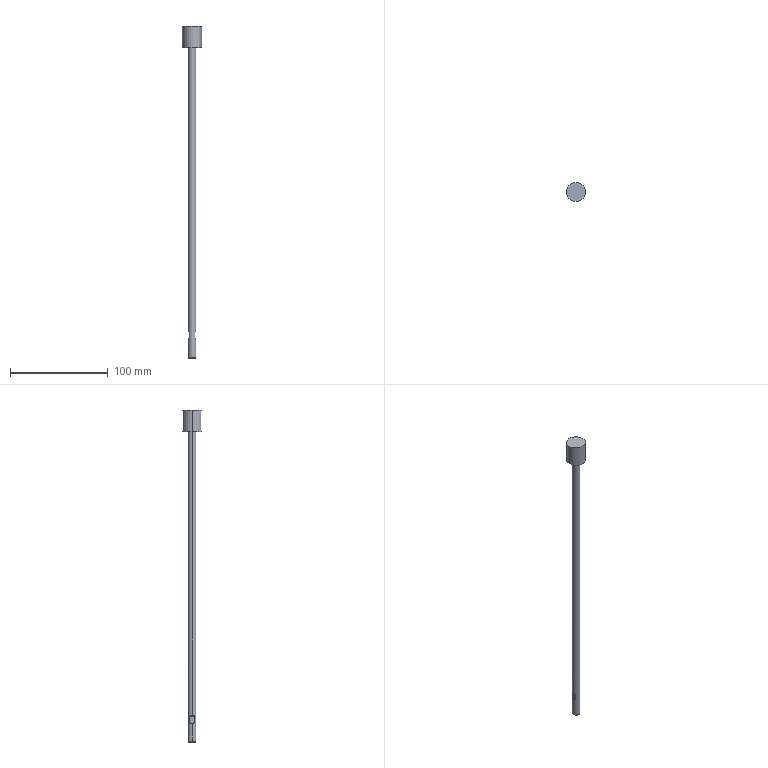Component | SolidWorks | F01AE00111-A2000-21TopEdgeAssembly-1_MA20x250SU(0)+(CS1-M-2)-1_20UMA250 Rod-1 | 1 solid | 15 faces | box 19.5 x 19.5 x 339 mm | volume 22445 mm3 | plane 9 | cylinder 4 | cone 2 | commonest cylinder face diameters 19.5 x2 8 x2
build123d program:
from build123d import *

# Parameters (mm, degrees)
CUT_EXTRUDE1_DEPTH      = 3
CUT_EXTRUDE1_DEPTH_BACK = 3


with BuildPart() as part:
    # Sketch1 → Revolve1 (revolve)
    with BuildSketch(Plane.XY, mode=Mode.PRIVATE) as revolve1_sk:
        Polygon((0, 0), (0, 3.233), (0.767, 4), (317, 4), (317, 9.75), (339, 9.75), (339, 0), align=None)
    revolve(revolve1_sk.sketch.rotate(Axis((339, 0, 0), (-1, 0, 0)), 270), axis=Axis((339, 0, 0), (-1, 0, 0)))

    # Sketch2 → Cut-Extrude1 (cut, two sides: drawn at the far end of the back side and taken through both)
    with BuildSketch(Plane(origin=(0, 0, 0), x_dir=(1, 0, 0), z_dir=(0, 1, 0)).offset(-CUT_EXTRUDE1_DEPTH_BACK)):
        Polygon((-5, 12), (-5, -12), (35.4, -12), (26.4, -3), (20, -3), (18, -5), (18, -10), (-3, -10), (-3, 10), (18, 10), (18, 5), (20, 3), (26.4, 3), (35.4, 12), align=None)
    extrude(amount=CUT_EXTRUDE1_DEPTH + CUT_EXTRUDE1_DEPTH_BACK, mode=Mode.SUBTRACT)


solid = part.part

# Placed as in the assembly
solid = solid.moved(Location((-109.352, 82.548, -371.975), (0, -90, 0)))
STEP:
#1=COLOUR_RGB('',0.7922,0.8196,0.9333);
#2=FILL_AREA_STYLE_COLOUR('',#1);
#3=FILL_AREA_STYLE('',(#2));
#4=SURFACE_STYLE_FILL_AREA(#3);
#5=SURFACE_SIDE_STYLE('',(#4));
#6=SURFACE_STYLE_USAGE(.BOTH.,#5);
#7=PRESENTATION_STYLE_ASSIGNMENT((#6));
#8=CARTESIAN_POINT('',(-3.921,3.25,-1.298));
#9=VERTEX_POINT('',#8);
#10=CARTESIAN_POINT('',(-4.689,3.25,-1.298));
#11=VERTEX_POINT('',#10);
#12=CARTESIAN_POINT('',(-4.305,3.25,-1.298));
#13=DIRECTION('',(-0.,-0.,-1.));
#14=DIRECTION('',(1.,0.,0.));
#15=AXIS2_PLACEMENT_3D('',#12,#13,#14);
#16=CIRCLE('',#15,0.3839);
#17=EDGE_CURVE('',#9,#11,#16,.T.);
#18=ORIENTED_EDGE('',*,*,#17,.T.);
#19=CARTESIAN_POINT('',(-4.689,3.25,-2.164));
#20=VERTEX_POINT('',#19);
#21=CARTESIAN_POINT('',(-4.689,3.25,-1.298));
#22=DIRECTION('',(-0.,-0.,-1.));
#23=VECTOR('',#22,39.37);
#24=LINE('',#21,#23);
#25=EDGE_CURVE('',#11,#20,#24,.T.);
#26=ORIENTED_EDGE('',*,*,#25,.T.);
#27=CARTESIAN_POINT('',(-3.921,3.25,-2.164));
#28=VERTEX_POINT('',#27);
#29=CARTESIAN_POINT('',(-4.305,3.25,-2.164));
#30=DIRECTION('',(-0.,-0.,-1.));
#31=DIRECTION('',(1.,0.,0.));
#32=AXIS2_PLACEMENT_3D('',#29,#30,#31);
#33=CIRCLE('',#32,0.3839);
#34=EDGE_CURVE('',#28,#20,#33,.T.);
#35=ORIENTED_EDGE('',*,*,#34,.F.);
#36=CARTESIAN_POINT('',(-3.921,3.25,-1.298));
#37=DIRECTION('',(-0.,-0.,-1.));
#38=VECTOR('',#37,39.37);
#39=LINE('',#36,#38);
#40=EDGE_CURVE('',#9,#28,#39,.T.);
#41=ORIENTED_EDGE('',*,*,#40,.F.);
#42=EDGE_LOOP('',(#18,#26,#35,#41));
#43=FACE_OUTER_BOUND('',#42,.T.);
#44=CARTESIAN_POINT('',(-4.305,3.25,-1.298));
#45=DIRECTION('',(-0.,-0.,-1.));
#46=DIRECTION('',(1.,0.,0.));
#47=AXIS2_PLACEMENT_3D('',#44,#45,#46);
#48=CYLINDRICAL_SURFACE('',#47,0.3839);
#49=ADVANCED_FACE('',(#43),#48,.T.);
#50=CARTESIAN_POINT('',(-4.148,3.25,-2.164));
#51=VERTEX_POINT('',#50);
#52=CARTESIAN_POINT('',(-4.463,3.25,-2.164));
#53=VERTEX_POINT('',#52);
#54=CARTESIAN_POINT('',(-4.305,3.25,-2.164));
#55=DIRECTION('',(-0.,-0.,-1.));
#56=DIRECTION('',(1.,0.,0.));
#57=AXIS2_PLACEMENT_3D('',#54,#55,#56);
#58=CIRCLE('',#57,0.1575);
#59=EDGE_CURVE('',#51,#53,#58,.T.);
#60=ORIENTED_EDGE('',*,*,#59,.T.);
#61=CARTESIAN_POINT('',(-4.463,3.25,-13.566));
#62=VERTEX_POINT('',#61);
#63=CARTESIAN_POINT('',(-4.463,3.25,-1.298));
#64=DIRECTION('',(-0.,-0.,-1.));
#65=VECTOR('',#64,39.37);
#66=LINE('',#63,#65);
#67=EDGE_CURVE('',#53,#62,#66,.T.);
#68=ORIENTED_EDGE('',*,*,#67,.T.);
#69=CARTESIAN_POINT('',(-4.423,3.146,-13.605));
#70=VERTEX_POINT('',#69);
#71=CARTESIAN_POINT('',(-4.463,3.25,-13.566));
#72=CARTESIAN_POINT('',(-4.463,3.211,-13.566));
#73=CARTESIAN_POINT('',(-4.449,3.175,-13.58));
#74=CARTESIAN_POINT('',(-4.423,3.146,-13.605));
#75=(BOUNDED_CURVE()B_SPLINE_CURVE(3,(#71,#72,#73,#74),.UNSPECIFIED.,.F.,.T.)B_SPLINE_CURVE_WITH_KNOTS((4,4),(3.142,3.864),.UNSPECIFIED.)CURVE()GEOMETRIC_REPRESENTATION_ITEM()RATIONAL_B_SPLINE_CURVE((1.,0.9569,0.9569,1.))REPRESENTATION_ITEM(''));
#76=EDGE_CURVE('',#62,#70,#75,.T.);
#77=ORIENTED_EDGE('',*,*,#76,.T.);
#78=CARTESIAN_POINT('',(-4.423,3.146,-13.857));
#79=VERTEX_POINT('',#78);
#80=CARTESIAN_POINT('',(-4.423,3.146,-1.298));
#81=DIRECTION('',(-0.,-0.,-1.));
#82=VECTOR('',#81,39.37);
#83=LINE('',#80,#82);
#84=EDGE_CURVE('',#70,#79,#83,.T.);
#85=ORIENTED_EDGE('',*,*,#84,.T.);
#86=CARTESIAN_POINT('',(-4.463,3.25,-13.897));
#87=VERTEX_POINT('',#86);
#88=CARTESIAN_POINT('',(-4.423,3.146,-13.857));
#89=CARTESIAN_POINT('',(-4.449,3.175,-13.883));
#90=CARTESIAN_POINT('',(-4.463,3.211,-13.897));
#91=CARTESIAN_POINT('',(-4.463,3.25,-13.897));
#92=(BOUNDED_CURVE()B_SPLINE_CURVE(3,(#88,#89,#90,#91),.UNSPECIFIED.,.F.,.T.)B_SPLINE_CURVE_WITH_KNOTS((4,4),(5.56,6.283),.UNSPECIFIED.)CURVE()GEOMETRIC_REPRESENTATION_ITEM()RATIONAL_B_SPLINE_CURVE((1.,0.9569,0.9569,1.))REPRESENTATION_ITEM(''));
#93=EDGE_CURVE('',#79,#87,#92,.T.);
#94=ORIENTED_EDGE('',*,*,#93,.T.);
#95=CARTESIAN_POINT('',(-4.463,3.25,-14.614));
#96=VERTEX_POINT('',#95);
#97=CARTESIAN_POINT('',(-4.463,3.25,-1.298));
#98=DIRECTION('',(-0.,-0.,-1.));
#99=VECTOR('',#98,39.37);
#100=LINE('',#97,#99);
#101=EDGE_CURVE('',#87,#96,#100,.T.);
#102=ORIENTED_EDGE('',*,*,#101,.T.);
#103=CARTESIAN_POINT('',(-4.148,3.25,-14.614));
#104=VERTEX_POINT('',#103);
#105=CARTESIAN_POINT('',(-4.305,3.25,-14.614));
#106=DIRECTION('',(-0.,-0.,-1.));
#107=DIRECTION('',(1.,0.,0.));
#108=AXIS2_PLACEMENT_3D('',#105,#106,#107);
#109=CIRCLE('',#108,0.1575);
#110=EDGE_CURVE('',#104,#96,#109,.T.);
#111=ORIENTED_EDGE('',*,*,#110,.F.);
#112=CARTESIAN_POINT('',(-4.148,3.25,-13.897));
#113=VERTEX_POINT('',#112);
#114=CARTESIAN_POINT('',(-4.148,3.25,-1.298));
#115=DIRECTION('',(-0.,-0.,-1.));
#116=VECTOR('',#115,39.37);
#117=LINE('',#114,#116);
#118=EDGE_CURVE('',#113,#104,#117,.T.);
#119=ORIENTED_EDGE('',*,*,#118,.F.);
#120=CARTESIAN_POINT('',(-4.187,3.146,-13.857));
#121=VERTEX_POINT('',#120);
#122=CARTESIAN_POINT('',(-4.148,3.25,-13.897));
#123=CARTESIAN_POINT('',(-4.148,3.211,-13.897));
#124=CARTESIAN_POINT('',(-4.161,3.175,-13.883));
#125=CARTESIAN_POINT('',(-4.187,3.146,-13.857));
#126=(BOUNDED_CURVE()B_SPLINE_CURVE(3,(#122,#123,#124,#125),.UNSPECIFIED.,.F.,.T.)B_SPLINE_CURVE_WITH_KNOTS((4,4),(0.,0.7227),.UNSPECIFIED.)CURVE()GEOMETRIC_REPRESENTATION_ITEM()RATIONAL_B_SPLINE_CURVE((1.,0.9569,0.9569,1.))REPRESENTATION_ITEM(''));
#127=EDGE_CURVE('',#113,#121,#126,.T.);
#128=ORIENTED_EDGE('',*,*,#127,.T.);
#129=CARTESIAN_POINT('',(-4.187,3.146,-13.605));
#130=VERTEX_POINT('',#129);
#131=CARTESIAN_POINT('',(-4.187,3.146,-1.298));
#132=DIRECTION('',(0.,0.,1.));
#133=VECTOR('',#132,39.37);
#134=LINE('',#131,#133);
#135=EDGE_CURVE('',#121,#130,#134,.T.);
#136=ORIENTED_EDGE('',*,*,#135,.T.);
#137=CARTESIAN_POINT('',(-4.148,3.25,-13.566));
#138=VERTEX_POINT('',#137);
#139=CARTESIAN_POINT('',(-4.187,3.146,-13.605));
#140=CARTESIAN_POINT('',(-4.161,3.175,-13.58));
#141=CARTESIAN_POINT('',(-4.148,3.211,-13.566));
#142=CARTESIAN_POINT('',(-4.148,3.25,-13.566));
#143=(BOUNDED_CURVE()B_SPLINE_CURVE(3,(#139,#140,#141,#142),.UNSPECIFIED.,.F.,.T.)B_SPLINE_CURVE_WITH_KNOTS((4,4),(2.419,3.142),.UNSPECIFIED.)CURVE()GEOMETRIC_REPRESENTATION_ITEM()RATIONAL_B_SPLINE_CURVE((1.,0.9569,0.9569,1.))REPRESENTATION_ITEM(''));
#144=EDGE_CURVE('',#130,#138,#143,.T.);
#145=ORIENTED_EDGE('',*,*,#144,.T.);
#146=CARTESIAN_POINT('',(-4.148,3.25,-1.298));
#147=DIRECTION('',(-0.,-0.,-1.));
#148=VECTOR('',#147,39.37);
#149=LINE('',#146,#148);
#150=EDGE_CURVE('',#51,#138,#149,.T.);
#151=ORIENTED_EDGE('',*,*,#150,.F.);
#152=EDGE_LOOP('',(#60,#68,#77,#85,#94,#102,#111,#119,#128,#136,#145,#151));
#153=FACE_OUTER_BOUND('',#152,.T.);
#154=CARTESIAN_POINT('',(-4.305,3.25,-1.298));
#155=DIRECTION('',(-0.,-0.,-1.));
#156=DIRECTION('',(1.,0.,0.));
#157=AXIS2_PLACEMENT_3D('',#154,#155,#156);
#158=CYLINDRICAL_SURFACE('',#157,0.1575);
#159=ADVANCED_FACE('',(#153),#158,.T.);
#160=CARTESIAN_POINT('',(-4.178,3.25,-14.645));
#161=VERTEX_POINT('',#160);
#162=CARTESIAN_POINT('',(-4.432,3.25,-14.645));
#163=VERTEX_POINT('',#162);
#164=CARTESIAN_POINT('',(-4.305,3.25,-14.645));
#165=DIRECTION('',(-0.,-0.,-1.));
#166=DIRECTION('',(1.,0.,0.));
#167=AXIS2_PLACEMENT_3D('',#164,#165,#166);
#168=CIRCLE('',#167,0.1273);
#169=EDGE_CURVE('',#161,#163,#168,.T.);
#170=ORIENTED_EDGE('',*,*,#169,.F.);
#171=CARTESIAN_POINT('',(-4.148,3.25,-14.614));
#172=DIRECTION('',(0.7071,-0.,0.7071));
#173=VECTOR('',#172,39.37);
#174=LINE('',#171,#173);
#175=EDGE_CURVE('',#161,#104,#174,.T.);
#176=ORIENTED_EDGE('',*,*,#175,.T.);
#177=ORIENTED_EDGE('',*,*,#110,.T.);
#178=CARTESIAN_POINT('',(-4.463,3.25,-14.614));
#179=DIRECTION('',(-0.7071,0.,0.7071));
#180=VECTOR('',#179,39.37);
#181=LINE('',#178,#180);
#182=EDGE_CURVE('',#163,#96,#181,.T.);
#183=ORIENTED_EDGE('',*,*,#182,.F.);
#184=EDGE_LOOP('',(#170,#176,#177,#183));
#185=FACE_OUTER_BOUND('',#184,.T.);
#186=CARTESIAN_POINT('',(-4.305,3.25,-14.614));
#187=DIRECTION('',(0.,0.,1.));
#188=DIRECTION('',(-1.,0.,0.));
#189=AXIS2_PLACEMENT_3D('',#186,#187,#188);
#190=CONICAL_SURFACE('',#189,0.1575,0.7854);
#191=ADVANCED_FACE('',(#185),#190,.T.);
#192=CARTESIAN_POINT('',(-4.305,3.25,-14.645));
#193=DIRECTION('',(-0.,-0.,-1.));
#194=DIRECTION('',(1.,0.,0.));
#195=AXIS2_PLACEMENT_3D('',#192,#193,#194);
#196=CIRCLE('',#195,0.1273);
#197=EDGE_CURVE('',#163,#161,#196,.T.);
#198=ORIENTED_EDGE('',*,*,#197,.T.);
#199=ORIENTED_EDGE('',*,*,#169,.T.);
#200=EDGE_LOOP('',(#198,#199));
#201=FACE_OUTER_BOUND('',#200,.T.);
#202=CARTESIAN_POINT('',(-4.305,3.25,-14.645));
#203=DIRECTION('',(0.,0.,1.));
#204=DIRECTION('',(-1.,0.,0.));
#205=AXIS2_PLACEMENT_3D('',#202,#203,#204);
#206=PLANE('',#205);
#207=ADVANCED_FACE('',(#201),#206,.F.);
#208=ORIENTED_EDGE('',*,*,#175,.F.);
#209=ORIENTED_EDGE('',*,*,#197,.F.);
#210=ORIENTED_EDGE('',*,*,#182,.T.);
#211=CARTESIAN_POINT('',(-4.305,3.25,-14.614));
#212=DIRECTION('',(-0.,-0.,-1.));
#213=DIRECTION('',(1.,0.,0.));
#214=AXIS2_PLACEMENT_3D('',#211,#212,#213);
#215=CIRCLE('',#214,0.1575);
#216=EDGE_CURVE('',#96,#104,#215,.T.);
#217=ORIENTED_EDGE('',*,*,#216,.T.);
#218=EDGE_LOOP('',(#208,#209,#210,#217));
#219=FACE_OUTER_BOUND('',#218,.T.);
#220=CARTESIAN_POINT('',(-4.305,3.25,-14.614));
#221=DIRECTION('',(0.,0.,1.));
#222=DIRECTION('',(-1.,0.,0.));
#223=AXIS2_PLACEMENT_3D('',#220,#221,#222);
#224=CONICAL_SURFACE('',#223,0.1575,0.7854);
#225=ADVANCED_FACE('',(#219),#224,.T.);
#226=ORIENTED_EDGE('',*,*,#67,.F.);
#227=CARTESIAN_POINT('',(-4.305,3.25,-2.164));
#228=DIRECTION('',(-0.,-0.,-1.));
#229=DIRECTION('',(1.,0.,0.));
#230=AXIS2_PLACEMENT_3D('',#227,#228,#229);
#231=CIRCLE('',#230,0.1575);
#232=EDGE_CURVE('',#53,#51,#231,.T.);
#233=ORIENTED_EDGE('',*,*,#232,.T.);
#234=ORIENTED_EDGE('',*,*,#150,.T.);
#235=CARTESIAN_POINT('',(-4.187,3.354,-13.605));
#236=VERTEX_POINT('',#235);
#237=CARTESIAN_POINT('',(-4.148,3.25,-13.566));
#238=CARTESIAN_POINT('',(-4.148,3.289,-13.566));
#239=CARTESIAN_POINT('',(-4.161,3.325,-13.58));
#240=CARTESIAN_POINT('',(-4.187,3.354,-13.605));
#241=(BOUNDED_CURVE()B_SPLINE_CURVE(3,(#237,#238,#239,#240),.UNSPECIFIED.,.F.,.T.)B_SPLINE_CURVE_WITH_KNOTS((4,4),(3.142,3.864),.UNSPECIFIED.)CURVE()GEOMETRIC_REPRESENTATION_ITEM()RATIONAL_B_SPLINE_CURVE((1.,0.9569,0.9569,1.))REPRESENTATION_ITEM(''));
#242=EDGE_CURVE('',#138,#236,#241,.T.);
#243=ORIENTED_EDGE('',*,*,#242,.T.);
#244=CARTESIAN_POINT('',(-4.187,3.354,-13.857));
#245=VERTEX_POINT('',#244);
#246=CARTESIAN_POINT('',(-4.187,3.354,-1.298));
#247=DIRECTION('',(-0.,-0.,-1.));
#248=VECTOR('',#247,39.37);
#249=LINE('',#246,#248);
#250=EDGE_CURVE('',#236,#245,#249,.T.);
#251=ORIENTED_EDGE('',*,*,#250,.T.);
#252=CARTESIAN_POINT('',(-4.187,3.354,-13.857));
#253=CARTESIAN_POINT('',(-4.161,3.325,-13.883));
#254=CARTESIAN_POINT('',(-4.148,3.289,-13.897));
#255=CARTESIAN_POINT('',(-4.148,3.25,-13.897));
#256=(BOUNDED_CURVE()B_SPLINE_CURVE(3,(#252,#253,#254,#255),.UNSPECIFIED.,.F.,.T.)B_SPLINE_CURVE_WITH_KNOTS((4,4),(5.56,6.283),.UNSPECIFIED.)CURVE()GEOMETRIC_REPRESENTATION_ITEM()RATIONAL_B_SPLINE_CURVE((1.,0.9569,0.9569,1.))REPRESENTATION_ITEM(''));
#257=EDGE_CURVE('',#245,#113,#256,.T.);
#258=ORIENTED_EDGE('',*,*,#257,.T.);
#259=ORIENTED_EDGE('',*,*,#118,.T.);
#260=ORIENTED_EDGE('',*,*,#216,.F.);
#261=ORIENTED_EDGE('',*,*,#101,.F.);
#262=CARTESIAN_POINT('',(-4.423,3.354,-13.857));
#263=VERTEX_POINT('',#262);
#264=CARTESIAN_POINT('',(-4.463,3.25,-13.897));
#265=CARTESIAN_POINT('',(-4.463,3.289,-13.897));
#266=CARTESIAN_POINT('',(-4.449,3.325,-13.883));
#267=CARTESIAN_POINT('',(-4.423,3.354,-13.857));
#268=(BOUNDED_CURVE()B_SPLINE_CURVE(3,(#264,#265,#266,#267),.UNSPECIFIED.,.F.,.T.)B_SPLINE_CURVE_WITH_KNOTS((4,4),(0.,0.7227),.UNSPECIFIED.)CURVE()GEOMETRIC_REPRESENTATION_ITEM()RATIONAL_B_SPLINE_CURVE((1.,0.9569,0.9569,1.))REPRESENTATION_ITEM(''));
#269=EDGE_CURVE('',#87,#263,#268,.T.);
#270=ORIENTED_EDGE('',*,*,#269,.T.);
#271=CARTESIAN_POINT('',(-4.423,3.354,-13.605));
#272=VERTEX_POINT('',#271);
#273=CARTESIAN_POINT('',(-4.423,3.354,-1.298));
#274=DIRECTION('',(0.,0.,1.));
#275=VECTOR('',#274,39.37);
#276=LINE('',#273,#275);
#277=EDGE_CURVE('',#263,#272,#276,.T.);
#278=ORIENTED_EDGE('',*,*,#277,.T.);
#279=CARTESIAN_POINT('',(-4.423,3.354,-13.605));
#280=CARTESIAN_POINT('',(-4.449,3.325,-13.58));
#281=CARTESIAN_POINT('',(-4.463,3.289,-13.566));
#282=CARTESIAN_POINT('',(-4.463,3.25,-13.566));
#283=(BOUNDED_CURVE()B_SPLINE_CURVE(3,(#279,#280,#281,#282),.UNSPECIFIED.,.F.,.T.)B_SPLINE_CURVE_WITH_KNOTS((4,4),(2.419,3.142),.UNSPECIFIED.)CURVE()GEOMETRIC_REPRESENTATION_ITEM()RATIONAL_B_SPLINE_CURVE((1.,0.9569,0.9569,1.))REPRESENTATION_ITEM(''));
#284=EDGE_CURVE('',#272,#62,#283,.T.);
#285=ORIENTED_EDGE('',*,*,#284,.T.);
#286=EDGE_LOOP('',(#226,#233,#234,#243,#251,#258,#259,#260,#261,#270,#278,#285));
#287=FACE_OUTER_BOUND('',#286,.T.);
#288=CARTESIAN_POINT('',(-4.305,3.25,-1.298));
#289=DIRECTION('',(-0.,-0.,-1.));
#290=DIRECTION('',(1.,0.,0.));
#291=AXIS2_PLACEMENT_3D('',#288,#289,#290);
#292=CYLINDRICAL_SURFACE('',#291,0.1575);
#293=ADVANCED_FACE('',(#287),#292,.T.);
#294=ORIENTED_EDGE('',*,*,#59,.F.);
#295=ORIENTED_EDGE('',*,*,#232,.F.);
#296=EDGE_LOOP('',(#294,#295));
#297=FACE_BOUND('',#296,.T.);
#298=ORIENTED_EDGE('',*,*,#34,.T.);
#299=CARTESIAN_POINT('',(-4.305,3.25,-2.164));
#300=DIRECTION('',(-0.,-0.,-1.));
#301=DIRECTION('',(1.,0.,0.));
#302=AXIS2_PLACEMENT_3D('',#299,#300,#301);
#303=CIRCLE('',#302,0.3839);
#304=EDGE_CURVE('',#20,#28,#303,.T.);
#305=ORIENTED_EDGE('',*,*,#304,.T.);
#306=EDGE_LOOP('',(#298,#305));
#307=FACE_OUTER_BOUND('',#306,.T.);
#308=CARTESIAN_POINT('',(-4.305,3.092,-2.164));
#309=DIRECTION('',(0.,0.,1.));
#310=DIRECTION('',(-1.,0.,0.));
#311=AXIS2_PLACEMENT_3D('',#308,#309,#310);
#312=PLANE('',#311);
#313=ADVANCED_FACE('',(#297,#307),#312,.F.);
#314=ORIENTED_EDGE('',*,*,#25,.F.);
#315=CARTESIAN_POINT('',(-4.305,3.25,-1.298));
#316=DIRECTION('',(-0.,-0.,-1.));
#317=DIRECTION('',(1.,0.,0.));
#318=AXIS2_PLACEMENT_3D('',#315,#316,#317);
#319=CIRCLE('',#318,0.3839);
#320=EDGE_CURVE('',#11,#9,#319,.T.);
#321=ORIENTED_EDGE('',*,*,#320,.T.);
#322=ORIENTED_EDGE('',*,*,#40,.T.);
#323=ORIENTED_EDGE('',*,*,#304,.F.);
#324=EDGE_LOOP('',(#314,#321,#322,#323));
#325=FACE_OUTER_BOUND('',#324,.T.);
#326=CARTESIAN_POINT('',(-4.305,3.25,-1.298));
#327=DIRECTION('',(-0.,-0.,-1.));
#328=DIRECTION('',(1.,0.,0.));
#329=AXIS2_PLACEMENT_3D('',#326,#327,#328);
#330=CYLINDRICAL_SURFACE('',#329,0.3839);
#331=ADVANCED_FACE('',(#325),#330,.T.);
#332=ORIENTED_EDGE('',*,*,#17,.F.);
#333=ORIENTED_EDGE('',*,*,#320,.F.);
#334=EDGE_LOOP('',(#332,#333));
#335=FACE_OUTER_BOUND('',#334,.T.);
#336=CARTESIAN_POINT('',(-4.305,2.866,-1.298));
#337=DIRECTION('',(-0.,-0.,-1.));
#338=DIRECTION('',(1.,-0.,-0.));
#339=AXIS2_PLACEMENT_3D('',#336,#337,#338);
#340=PLANE('',#339);
#341=ADVANCED_FACE('',(#335),#340,.F.);
#342=CARTESIAN_POINT('',(-4.187,3.368,-13.605));
#343=DIRECTION('',(-0.,-1.,0.));
#344=VECTOR('',#343,39.37);
#345=LINE('',#342,#344);
#346=EDGE_CURVE('',#236,#130,#345,.T.);
#347=ORIENTED_EDGE('',*,*,#346,.F.);
#348=ORIENTED_EDGE('',*,*,#242,.F.);
#349=ORIENTED_EDGE('',*,*,#144,.F.);
#350=EDGE_LOOP('',(#347,#348,#349));
#351=FACE_OUTER_BOUND('',#350,.T.);
#352=CARTESIAN_POINT('',(-3.833,3.368,-13.251));
#353=DIRECTION('',(-0.7071,0.,0.7071));
#354=DIRECTION('',(-0.7071,0.,-0.7071));
#355=AXIS2_PLACEMENT_3D('',#352,#353,#354);
#356=PLANE('',#355);
#357=ADVANCED_FACE('',(#351),#356,.F.);
#358=ORIENTED_EDGE('',*,*,#346,.T.);
#359=ORIENTED_EDGE('',*,*,#135,.F.);
#360=CARTESIAN_POINT('',(-4.187,3.368,-13.857));
#361=DIRECTION('',(-0.,-1.,0.));
#362=VECTOR('',#361,39.37);
#363=LINE('',#360,#362);
#364=EDGE_CURVE('',#245,#121,#363,.T.);
#365=ORIENTED_EDGE('',*,*,#364,.F.);
#366=ORIENTED_EDGE('',*,*,#250,.F.);
#367=EDGE_LOOP('',(#358,#359,#365,#366));
#368=FACE_OUTER_BOUND('',#367,.T.);
#369=CARTESIAN_POINT('',(-4.187,3.368,-13.605));
#370=DIRECTION('',(-1.,0.,0.));
#371=DIRECTION('',(-0.,-0.,-1.));
#372=AXIS2_PLACEMENT_3D('',#369,#370,#371);
#373=PLANE('',#372);
#374=ADVANCED_FACE('',(#368),#373,.F.);
#375=ORIENTED_EDGE('',*,*,#364,.T.);
#376=ORIENTED_EDGE('',*,*,#127,.F.);
#377=ORIENTED_EDGE('',*,*,#257,.F.);
#378=EDGE_LOOP('',(#375,#376,#377));
#379=FACE_OUTER_BOUND('',#378,.T.);
#380=CARTESIAN_POINT('',(-4.187,3.368,-13.857));
#381=DIRECTION('',(-0.7071,0.,-0.7071));
#382=DIRECTION('',(0.7071,-0.,-0.7071));
#383=AXIS2_PLACEMENT_3D('',#380,#381,#382);
#384=PLANE('',#383);
#385=ADVANCED_FACE('',(#379),#384,.F.);
#386=CARTESIAN_POINT('',(-4.423,3.368,-13.605));
#387=DIRECTION('',(-0.,-1.,0.));
#388=VECTOR('',#387,39.37);
#389=LINE('',#386,#388);
#390=EDGE_CURVE('',#272,#70,#389,.T.);
#391=ORIENTED_EDGE('',*,*,#390,.T.);
#392=ORIENTED_EDGE('',*,*,#76,.F.);
#393=ORIENTED_EDGE('',*,*,#284,.F.);
#394=EDGE_LOOP('',(#391,#392,#393));
#395=FACE_OUTER_BOUND('',#394,.T.);
#396=CARTESIAN_POINT('',(-4.423,3.368,-13.605));
#397=DIRECTION('',(0.7071,-0.,0.7071));
#398=DIRECTION('',(-0.7071,0.,0.7071));
#399=AXIS2_PLACEMENT_3D('',#396,#397,#398);
#400=PLANE('',#399);
#401=ADVANCED_FACE('',(#395),#400,.F.);
#402=ORIENTED_EDGE('',*,*,#390,.F.);
#403=ORIENTED_EDGE('',*,*,#277,.F.);
#404=CARTESIAN_POINT('',(-4.423,3.368,-13.857));
#405=DIRECTION('',(-0.,-1.,0.));
#406=VECTOR('',#405,39.37);
#407=LINE('',#404,#406);
#408=EDGE_CURVE('',#263,#79,#407,.T.);
#409=ORIENTED_EDGE('',*,*,#408,.T.);
#410=ORIENTED_EDGE('',*,*,#84,.F.);
#411=EDGE_LOOP('',(#402,#403,#409,#410));
#412=FACE_OUTER_BOUND('',#411,.T.);
#413=CARTESIAN_POINT('',(-4.423,3.368,-13.857));
#414=DIRECTION('',(1.,-0.,-0.));
#415=DIRECTION('',(0.,0.,1.));
#416=AXIS2_PLACEMENT_3D('',#413,#414,#415);
#417=PLANE('',#416);
#418=ADVANCED_FACE('',(#412),#417,.F.);
#419=ORIENTED_EDGE('',*,*,#408,.F.);
#420=ORIENTED_EDGE('',*,*,#269,.F.);
#421=ORIENTED_EDGE('',*,*,#93,.F.);
#422=EDGE_LOOP('',(#419,#420,#421));
#423=FACE_OUTER_BOUND('',#422,.T.);
#424=CARTESIAN_POINT('',(-4.502,3.368,-13.936));
#425=DIRECTION('',(0.7071,-0.,-0.7071));
#426=DIRECTION('',(0.7071,-0.,0.7071));
#427=AXIS2_PLACEMENT_3D('',#424,#425,#426);
#428=PLANE('',#427);
#429=ADVANCED_FACE('',(#423),#428,.F.);
#430=CLOSED_SHELL('',(#49,#159,#191,#207,#225,#293,#313,#331,#341,#357,#374,#385,#401,#418,#429));
#431=MANIFOLD_SOLID_BREP('',#430);
#432=STYLED_ITEM('',(#7),#431);
#433=(LENGTH_UNIT()NAMED_UNIT(*)SI_UNIT($,.METRE.));
#434=LENGTH_MEASURE_WITH_UNIT(LENGTH_MEASURE(0.0254),#433);
#435=DIMENSIONAL_EXPONENTS(1.,0.,0.,0.,0.,0.,0.);
#436=(CONVERSION_BASED_UNIT('',#434)LENGTH_UNIT()NAMED_UNIT(#435));
#437=UNCERTAINTY_MEASURE_WITH_UNIT(LENGTH_MEASURE(0.00001),#436,'','');
#438=(NAMED_UNIT(*)PLANE_ANGLE_UNIT()SI_UNIT($,.RADIAN.));
#439=(NAMED_UNIT(*)SI_UNIT($,.STERADIAN.)SOLID_ANGLE_UNIT());
#440=(GEOMETRIC_REPRESENTATION_CONTEXT(3)GLOBAL_UNCERTAINTY_ASSIGNED_CONTEXT((#437))GLOBAL_UNIT_ASSIGNED_CONTEXT((#436,#438,#439))REPRESENTATION_CONTEXT('',''));
#441=MECHANICAL_DESIGN_GEOMETRIC_PRESENTATION_REPRESENTATION('',(#432),#440);
#442=CARTESIAN_POINT('',(0.,0.,0.));
#443=DIRECTION('',(0.,0.,1.));
#444=DIRECTION('',(1.,0.,0.));
#445=AXIS2_PLACEMENT_3D('',#442,#443,#444);
#446=(LENGTH_UNIT()NAMED_UNIT(*)SI_UNIT($,.METRE.));
#447=LENGTH_MEASURE_WITH_UNIT(LENGTH_MEASURE(0.0254),#446);
#448=DIMENSIONAL_EXPONENTS(1.,0.,0.,0.,0.,0.,0.);
#449=(CONVERSION_BASED_UNIT('',#447)LENGTH_UNIT()NAMED_UNIT(#448));
#450=UNCERTAINTY_MEASURE_WITH_UNIT(LENGTH_MEASURE(0.00001),#449,'','');
#451=(NAMED_UNIT(*)PLANE_ANGLE_UNIT()SI_UNIT($,.RADIAN.));
#452=(NAMED_UNIT(*)SI_UNIT($,.STERADIAN.)SOLID_ANGLE_UNIT());
#453=(GEOMETRIC_REPRESENTATION_CONTEXT(3)GLOBAL_UNCERTAINTY_ASSIGNED_CONTEXT((#450))GLOBAL_UNIT_ASSIGNED_CONTEXT((#449,#451,#452))REPRESENTATION_CONTEXT('',''));
#454=ADVANCED_BREP_SHAPE_REPRESENTATION('',(#431,#445),#453);
#455=PRESENTATION_LAYER_ASSIGNMENT('','',(#432));